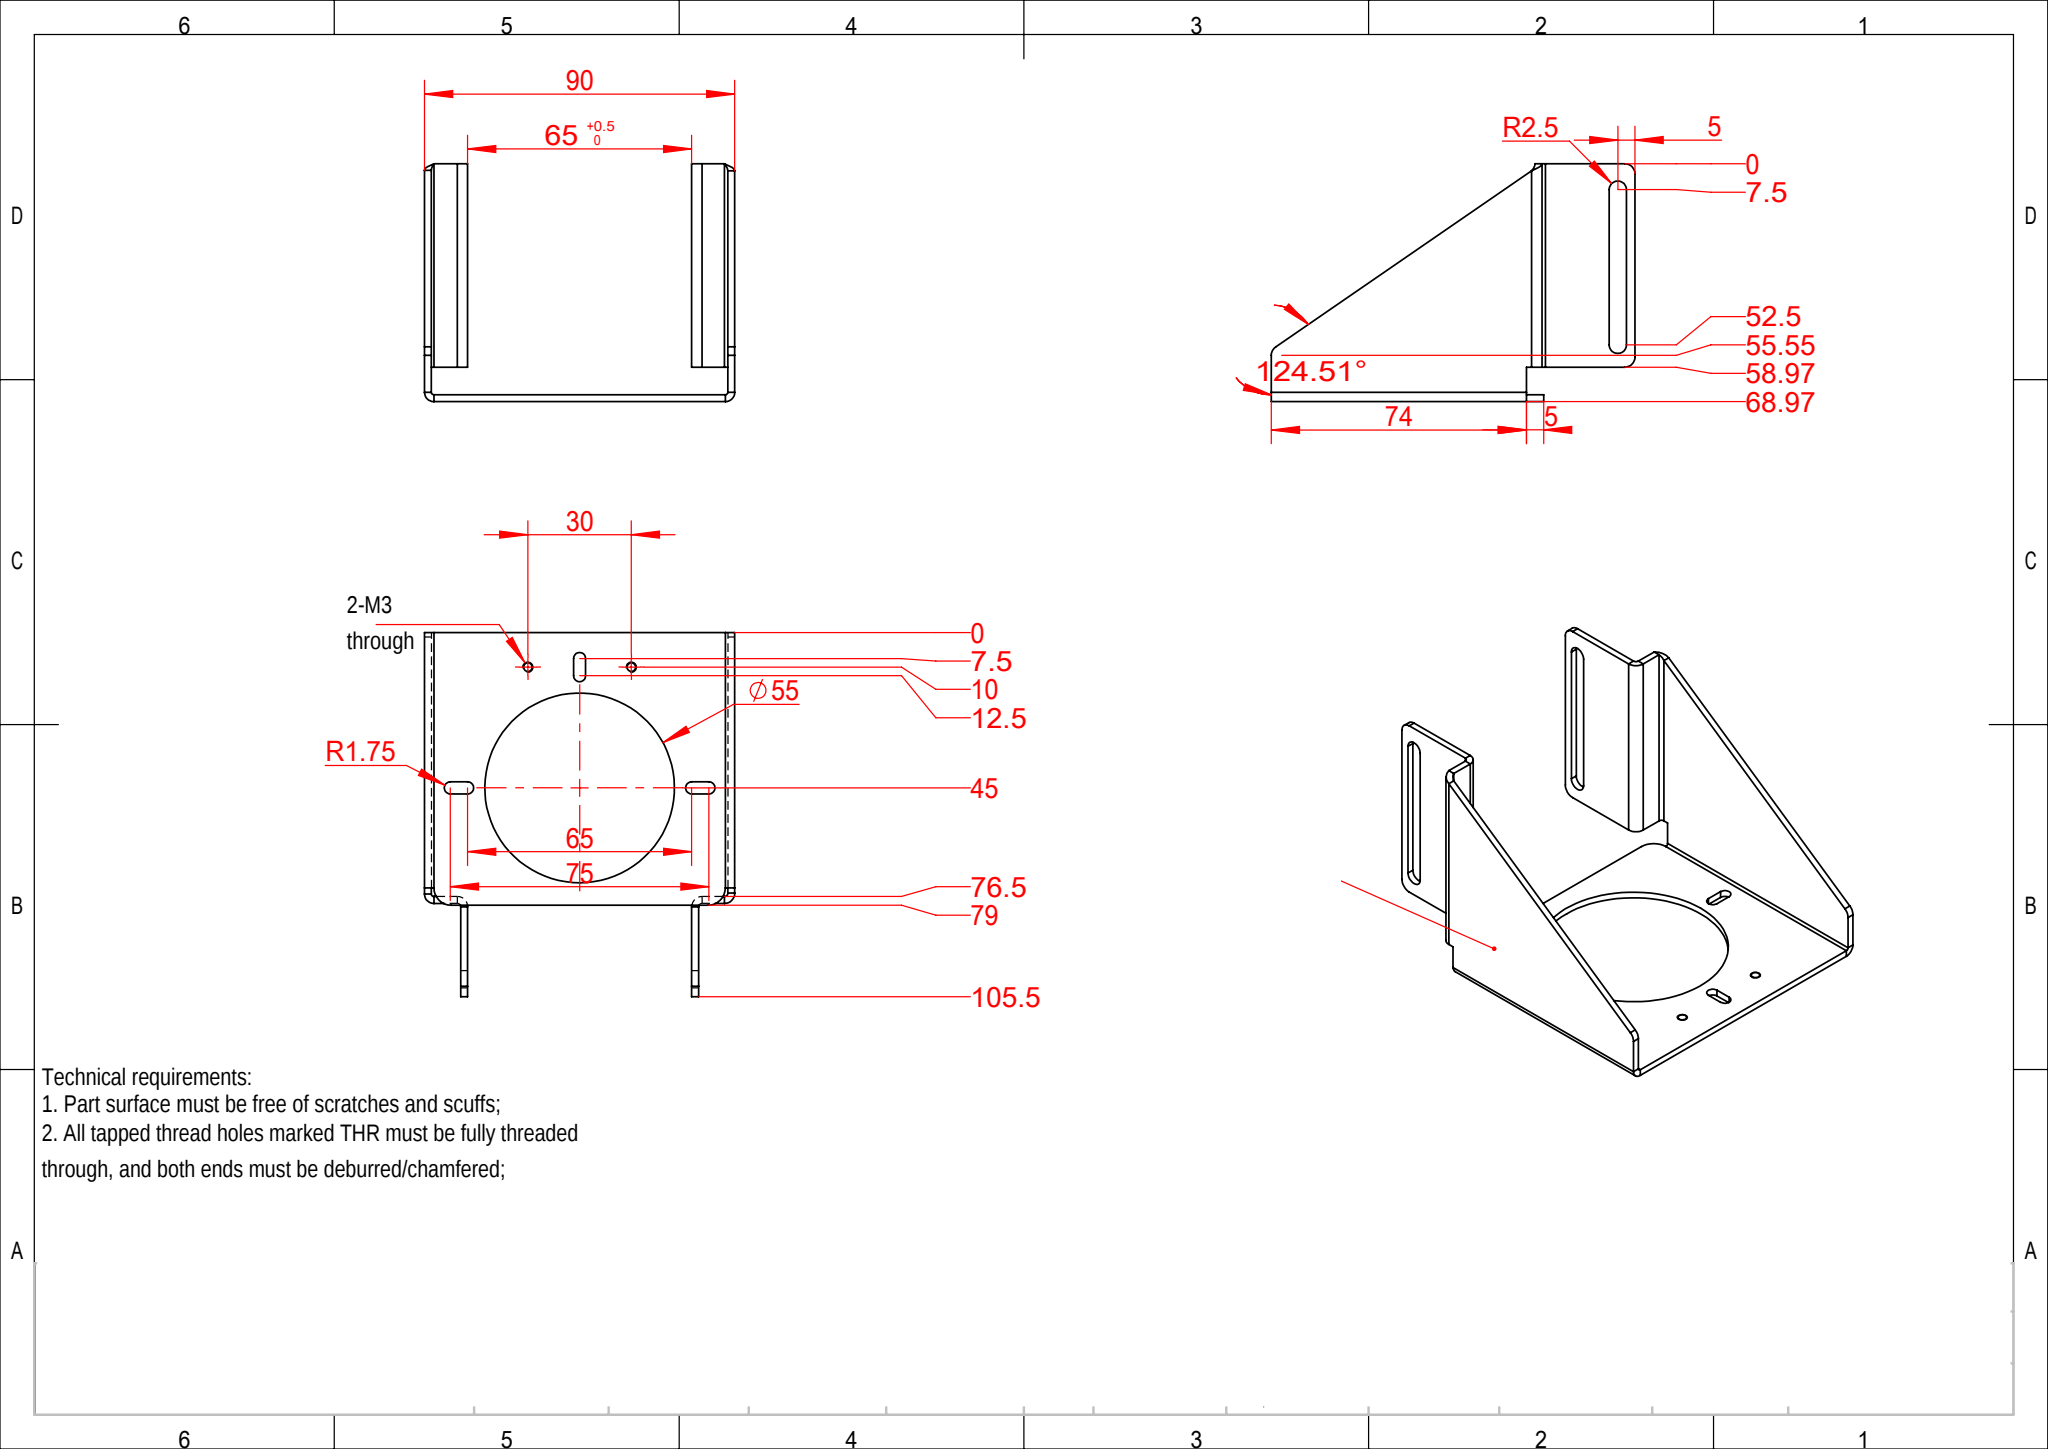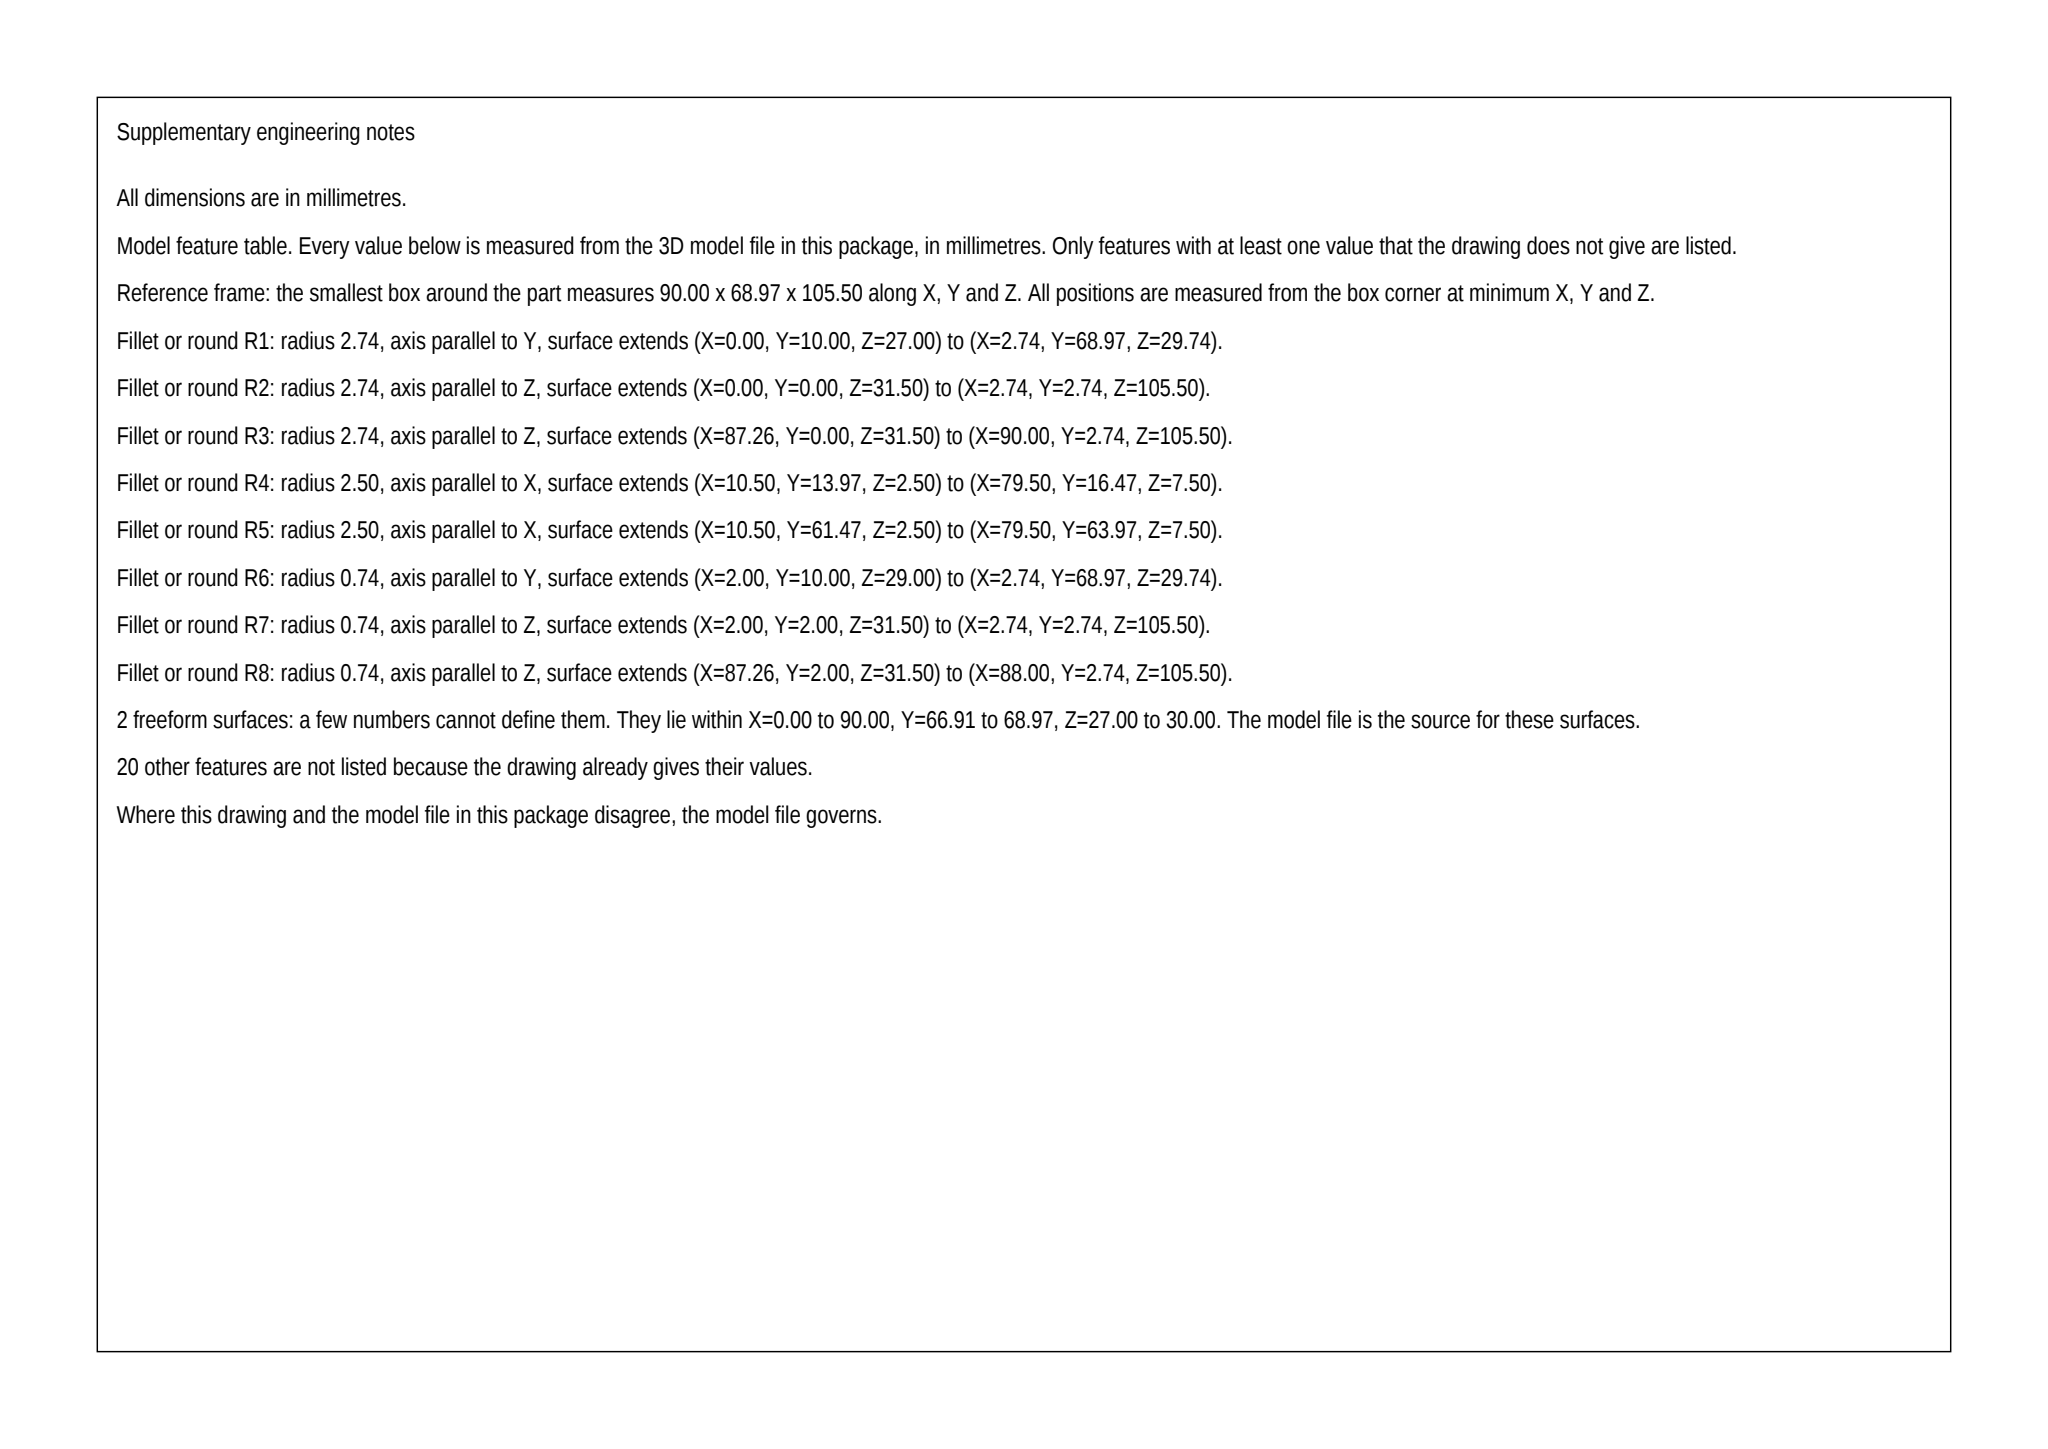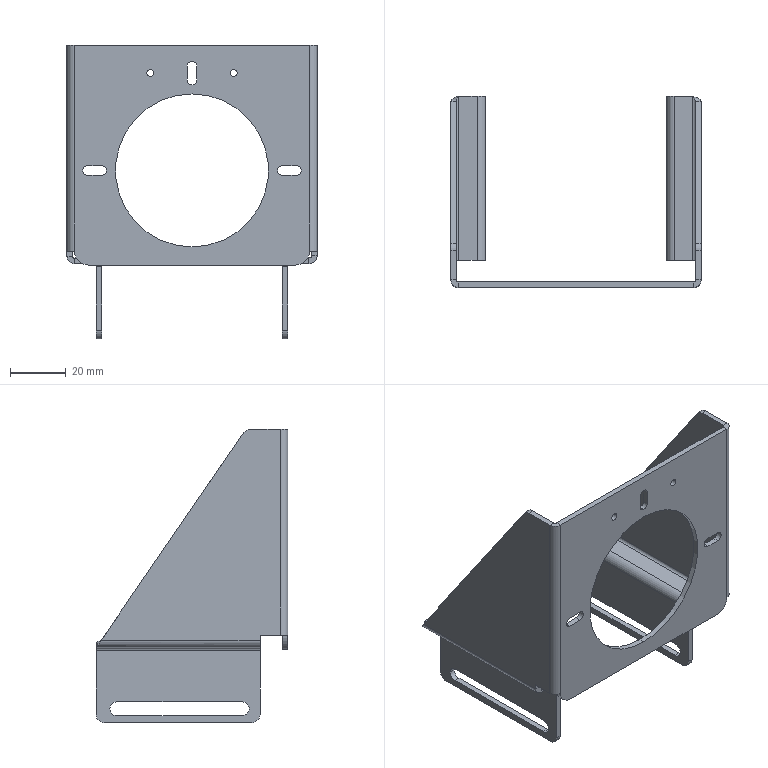Part | SolidWorks | mm | 1 solid | 95 faces | box 90 x 68.97 x 105.5 mm | volume 28858 mm3 | plane 54 | cylinder 39 | spline 2 | commonest cylinder face diameters 6 x9 3.5 x7 5 x6 2.5 x4 5.473 x3 1.473 x3 2 x3 55 x2